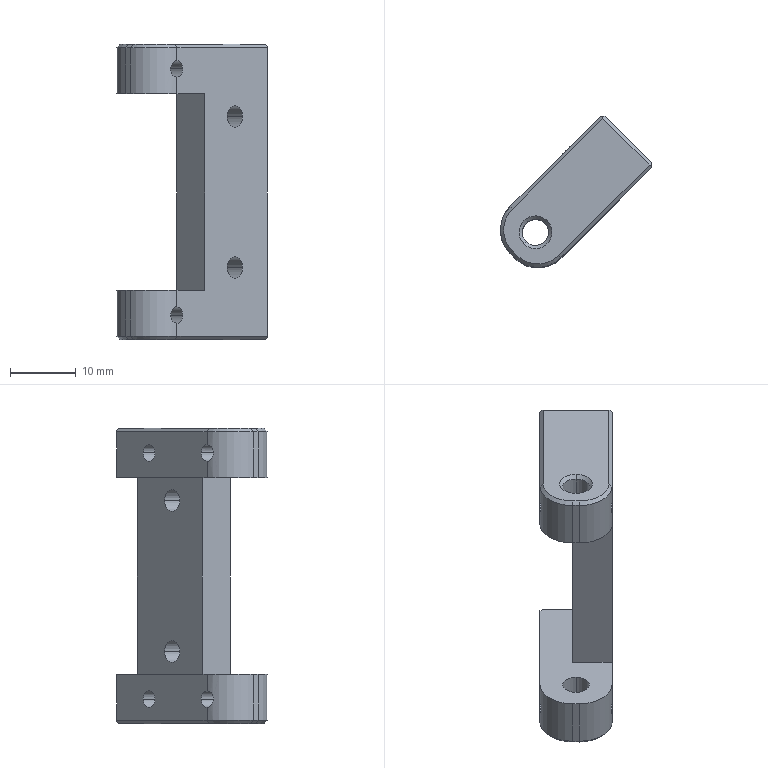Component | SolidWorks | GuideWheelFixedSeat-1 | 1 solid | 59 faces | volume 6019 mm3 | cylinder 24 | plane 23 | cone 12 | commonest cylinder face diameters 2.5 x12 3.3 x4 4 x4 10 x4